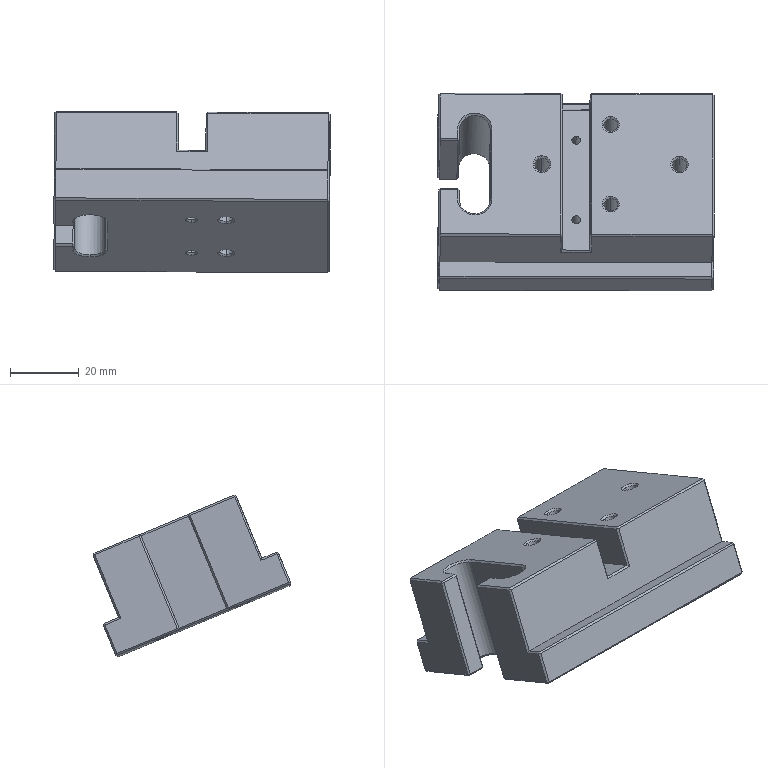Component | SolidWorks | 10-1 | 1 solid | 131 faces | box 80.19 x 57.47 x 46.93 mm | volume 99687 mm3 | plane 90 | cone 26 | cylinder 15 | commonest cylinder face diameters 2.5 x4 4 x4 4.2 x4 9 x3
build123d program:
from build123d import *

# Parameters (mm, degrees)
SKETCH1_W                 = 55
SKETCH1_H                 = 80
BOSS_EXTRUDE1_DEPTH       = 30
M5_TAPPED_HOLE1_D         = 4.2
M5_TAPPED_HOLE1_DEPTH     = 12.4
M5_TAPPED_HOLE1_TIP       = 1.262
SIZE_MM_DOWEL_PIN_HOLE1_D = 4
SKETCH6_W                 = 5
SKETCH6_H                 = 80
CUT_EXTRUDE1_DEPTH        = 20
CUT_EXTRUDE2_DEPTH        = 58.064
SKETCH8_W                 = 80
SKETCH8_H                 = 8
CUT_EXTRUDE3_DEPTH        = 12
M3_TAPPED_HOLE1_D         = 2.5
CHAMFER1_SIZE             = 0.5


with BuildPart() as part:
    # Sketch1 → Boss-Extrude1 (new body)
    with BuildSketch(Plane.XY):
        Rectangle(SKETCH1_W, SKETCH1_H)
    extrude(amount=BOSS_EXTRUDE1_DEPTH)

    # M5 Tapped Hole1
    with Locations(Plane.XY.offset(30)):
        with Locations((0, 30), (0, -10)):
            Hole(M5_TAPPED_HOLE1_D / 2, depth=M5_TAPPED_HOLE1_DEPTH)
            with Locations((0, 0, -(M5_TAPPED_HOLE1_DEPTH + M5_TAPPED_HOLE1_TIP / 2))):  # 118° drill point
                Cone(0, M5_TAPPED_HOLE1_D / 2, M5_TAPPED_HOLE1_TIP, mode=Mode.SUBTRACT)

    # Size mm Dowel Pin Hole1 (through all)
    with Locations(Plane.XY.offset(30)):
        with Locations((-12.5, 10), (12.5, 10)):
            Hole(SIZE_MM_DOWEL_PIN_HOLE1_D / 2)

    # Sketch6 → Cut-Extrude1 (cut)
    with BuildSketch(Plane.XY.offset(30)):
        with Locations((-25, 0)):
            Rectangle(SKETCH6_W, SKETCH6_H)
        with Locations((25, 0)):
            Rectangle(SKETCH6_W, SKETCH6_H)
    extrude(amount=-CUT_EXTRUDE1_DEPTH, mode=Mode.SUBTRACT)

    # Sketch7 → Cut-Extrude2 (cut, through all)
    with BuildSketch(Plane.XY.offset(30)):
        with BuildLine():
            Line((-7.5, -34), (-7.5, -46))
            Line((-7.5, -46), (7.5, -46))
            Line((7.5, -46), (7.5, -34))
            Line((7.5, -34), (11, -34))
            ThreePointArc((11, -34), (15.5, -29.5), (11, -25))
            Line((11, -25), (-11, -25))
            ThreePointArc((-11, -25), (-15.5, -29.5), (-11, -34))
            Line((-11, -34), (-7.5, -34))
        make_face()
    extrude(amount=-CUT_EXTRUDE2_DEPTH, mode=Mode.SUBTRACT)

    # Sketch8 → Cut-Extrude3 (cut)
    with BuildSketch(Plane.XY.offset(30)):
        Rectangle(SKETCH8_W, SKETCH8_H)
    extrude(amount=-CUT_EXTRUDE3_DEPTH, mode=Mode.SUBTRACT)

    # M3 Tapped Hole1 (through all)
    with Locations(Plane.XY.offset(18)):
        with Locations((-12.5, 0), (12.5, 0)):
            Hole(M3_TAPPED_HOLE1_D / 2)

    # Chamfer1
    chamfer1_edges = [part.edges().sort_by_distance(p)[0] for p in [
        (2.1, 30, 30),
        (14.5, 10, 30),
        (-10.5, 10, 30),
        (2.1, -10, 30),
        (14.5, 10, 0),
        (-10.5, 10, 0),
        (13.75, 0, 0),
        (-11.25, 0, 0),
        (-22.5, 22, 30),
        (-22.5, 40, 20),
        (0, 40, 30),
        (22.5, 22, 30),
        (0, 4, 30),
        (22.5, -22, 30),
        (15, -40, 30),
        (7.5, -37, 30),
        (9.25, -34, 30),
        (15.5, -29.5, 30),
        (0, -25, 30),
        (-15.5, -29.5, 30),
        (-9.25, -34, 30),
        (-7.5, -37, 30),
        (-15, -40, 30),
        (22.5, 4, 24),
        (22.5, 0, 18),
        (22.5, -4, 24),
        (0, -4, 30),
        (-22.5, 4, 24),
        (-22.5, 0, 18),
        (-22.5, -4, 24),
        (-22.5, -22, 30),
        (27.5, 0, 0),
        (0, 40, 0),
        (-27.5, 0, 0),
        (-22.5, -40, 20),
        (-25, -40, 10),
        (-27.5, 40, 5),
        (-27.5, 0, 10),
        (-27.5, -40, 5),
        (-17.5, -40, 0),
        (-7.5, -40, 15),
        (-7.5, -37, 0),
        (-7.5, -34, 15),
        (-9.25, -34, 0),
        (-15.5, -29.5, 0),
        (0, -25, 0),
        (15.5, -29.5, 0),
        (9.25, -34, 0),
        (7.5, -34, 15),
        (7.5, -37, 0),
        (7.5, -40, 15),
        (17.5, -40, 0),
        (22.5, -40, 20),
        (25, -40, 10),
        (27.5, 40, 5),
        (22.5, 40, 20),
        (25, 40, 10),
        (27.5, -40, 5),
        (27.5, 0, 10),
    ]]
    chamfer(chamfer1_edges, length=CHAMFER1_SIZE)


solid = part.part

# Placed as in the assembly
solid = solid.moved(Location((93.82, -79.908, 440.853), (-22.484, 0.3658, -89.992)))